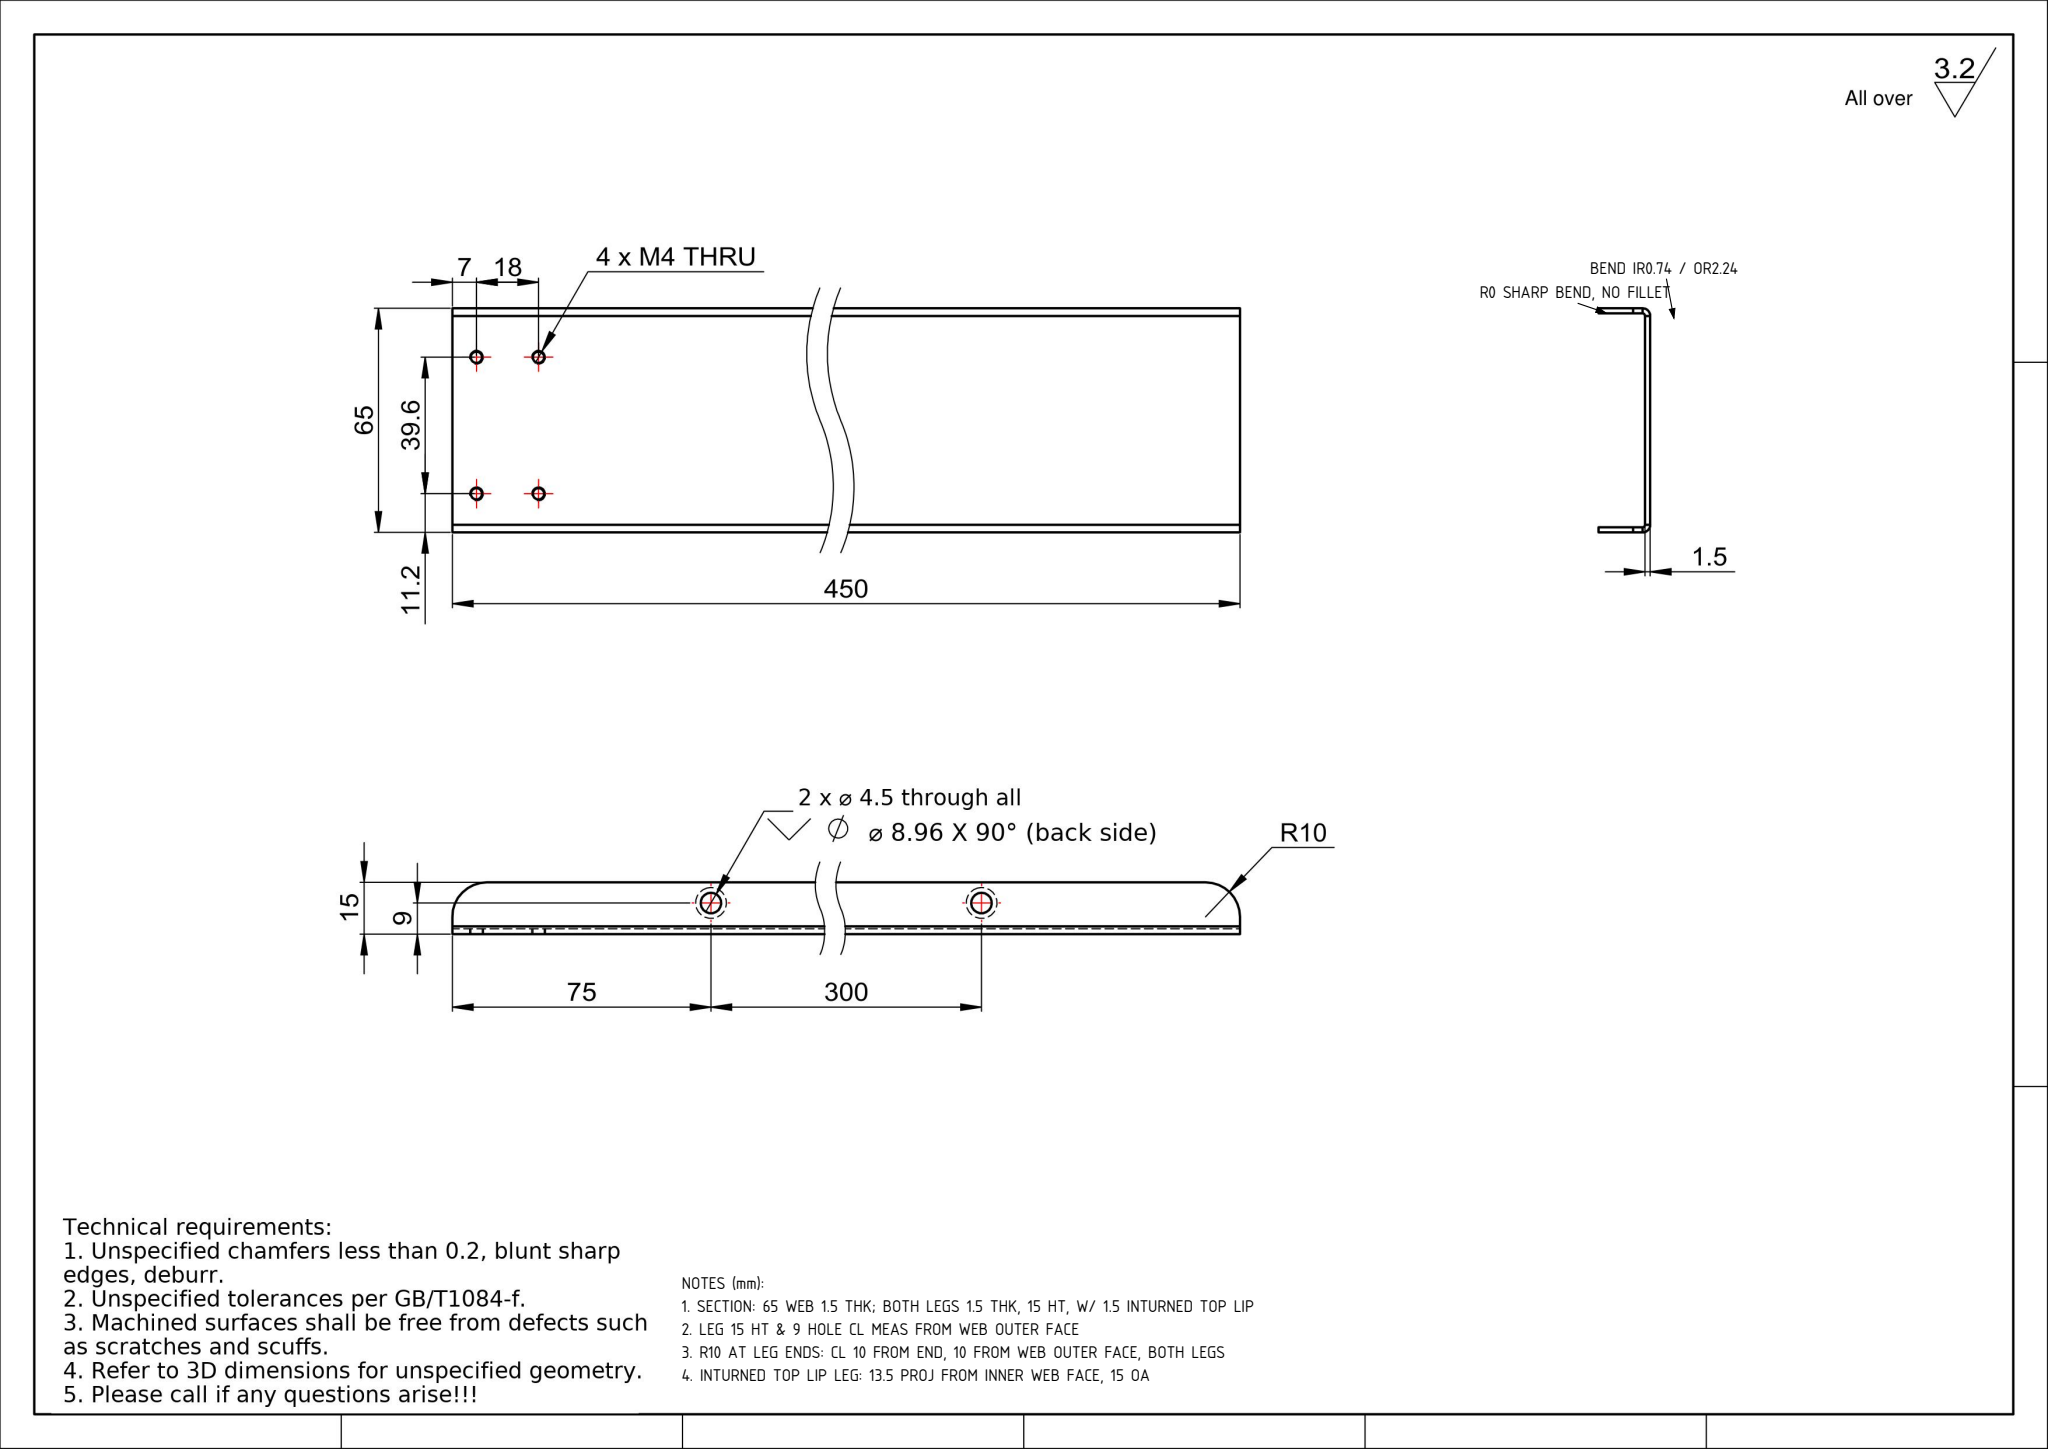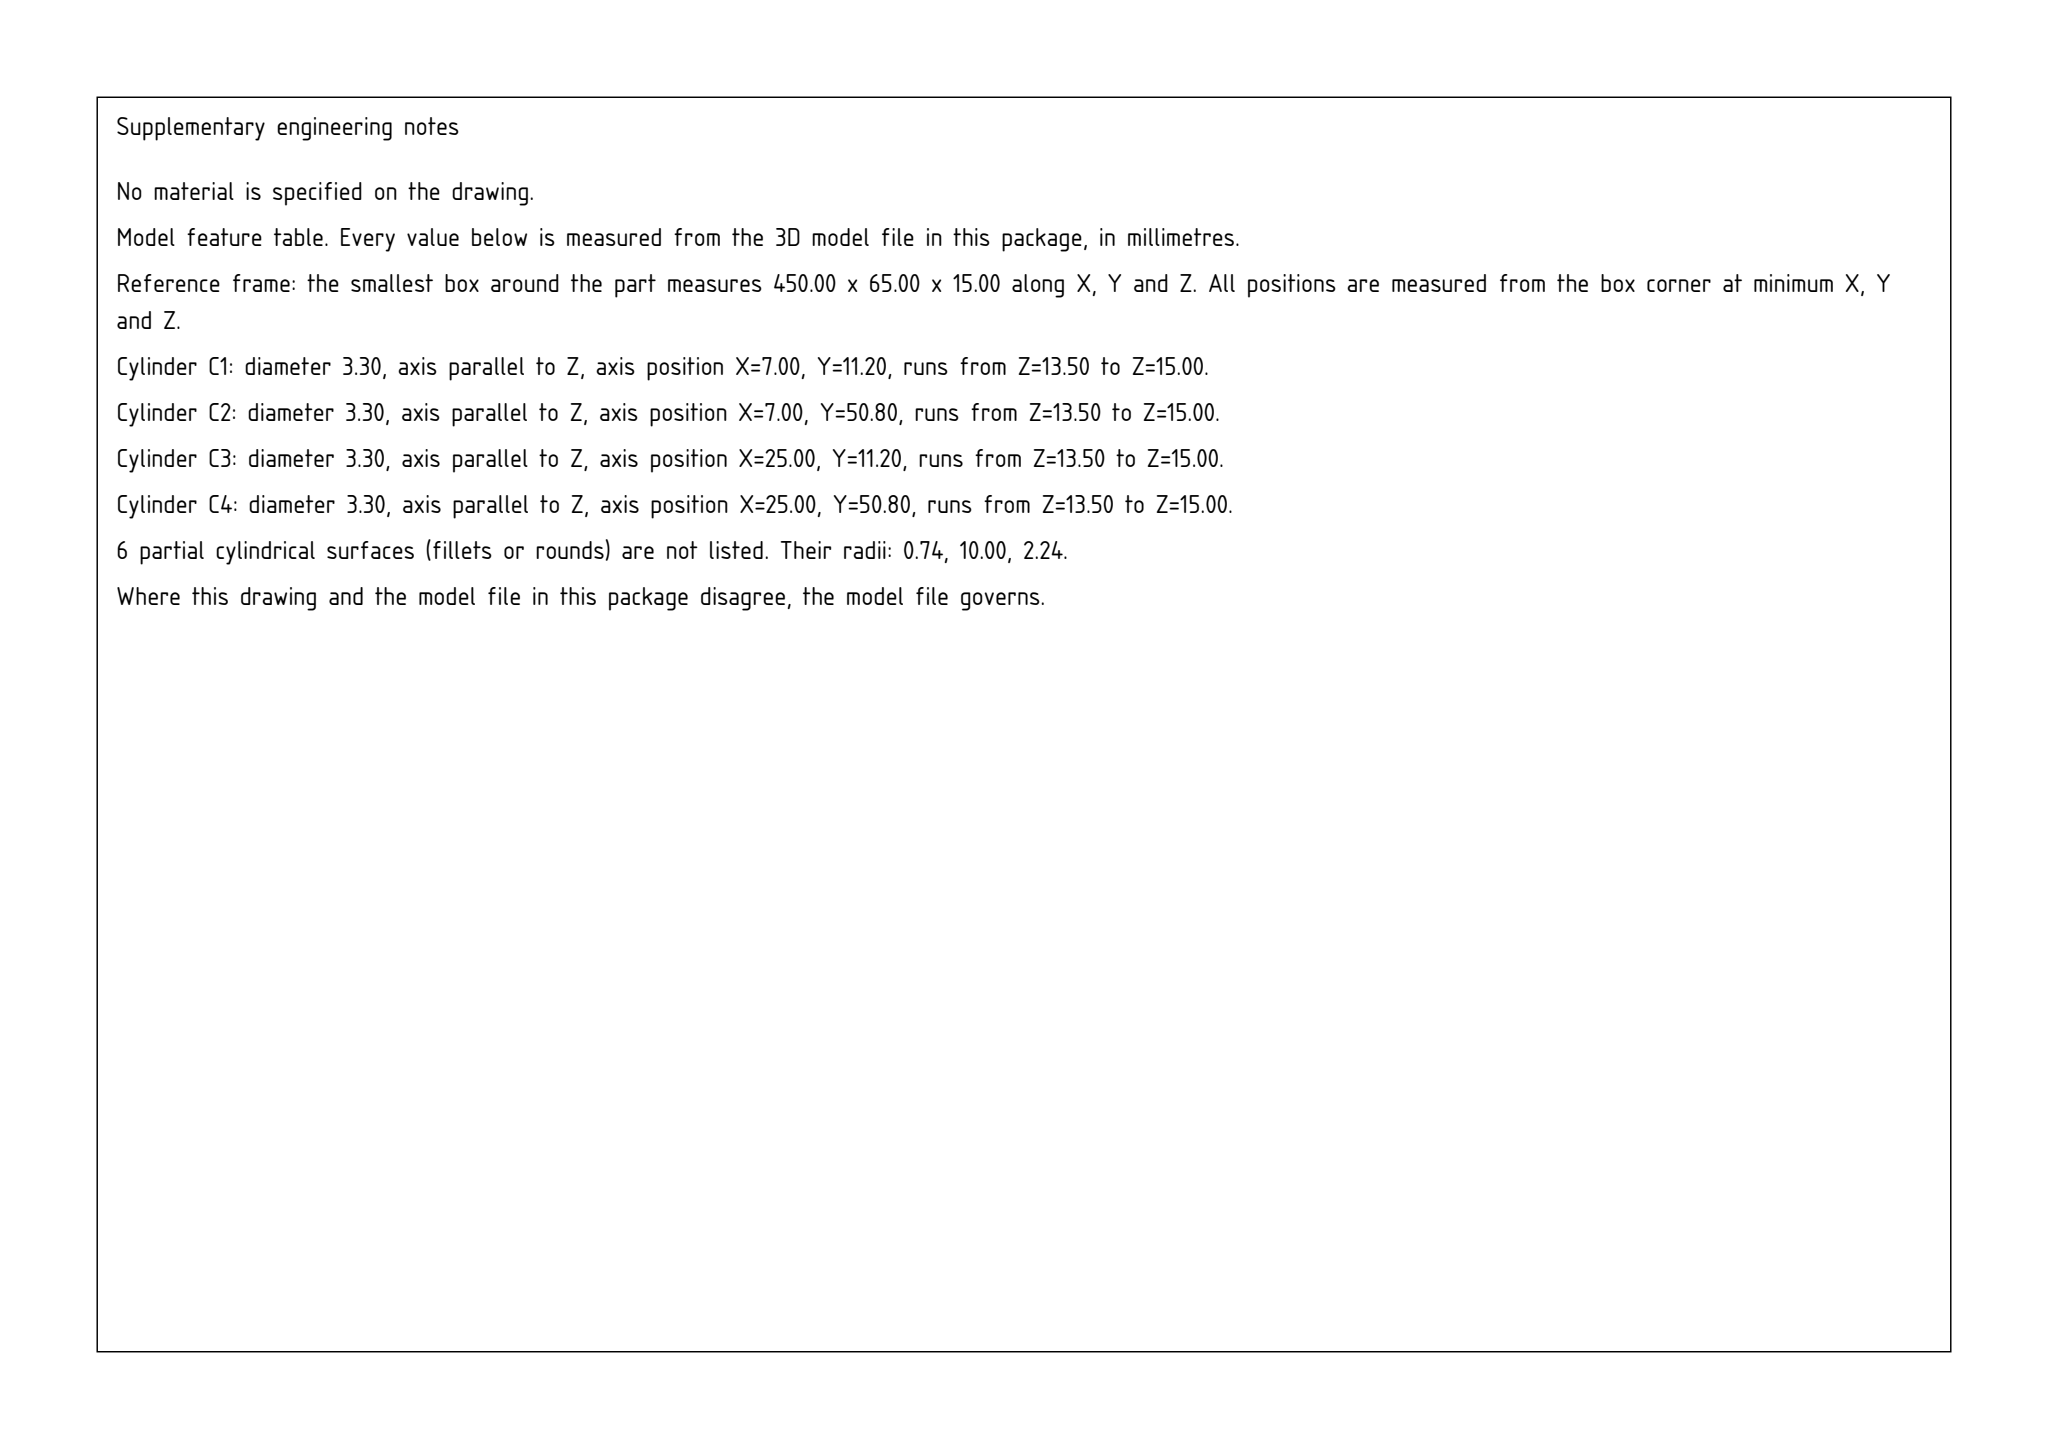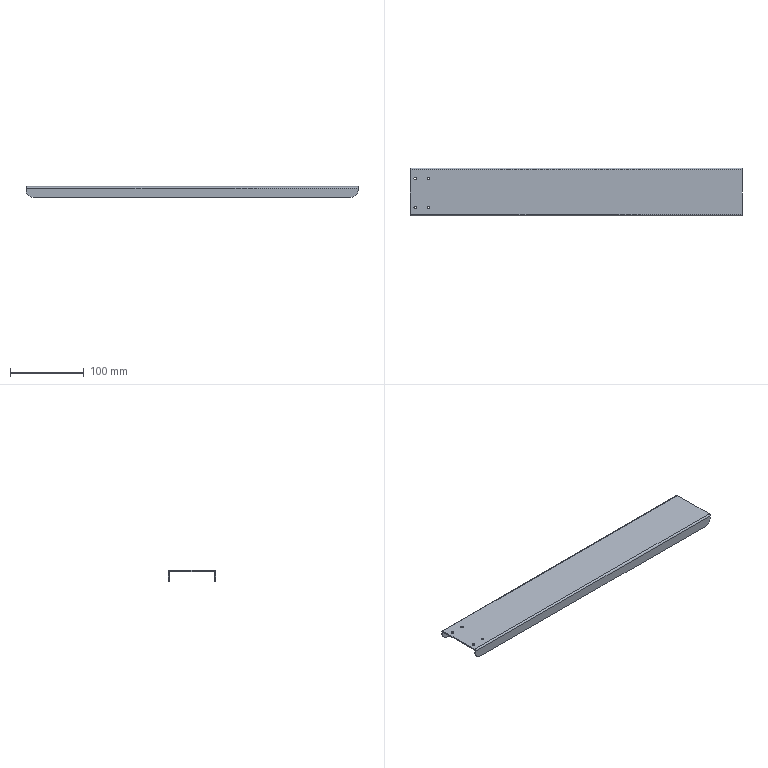Part | SolidWorks | mm | 1 solid | 38 faces | box 450 x 65 x 15 mm | volume 60926 mm3 | plane 18 | cylinder 16 | cone 4 | commonest cylinder face diameters 3.3 x8 20 x4 4.473 x2 1.473 x2
Drawing notes:
SECTION: 65 WEB 1.5 THK; BOTH LEGS 1.5 THK, 15 HT, W/ 1.5 INTURNED TOP LIP | from the solid: Y-planes 0/1.5 & 63.5/65 (1.5 thk legs); Z-planes 0, 13.5, 15; bbox 450x65x15
LEG 15 HT & 9 HOLE CL MEAS FROM WEB OUTER FACE | from the solid: Z-planes 0/15 give leg ht from web outer face at Z0; holes at z=9
LEG TO WEB BEND SHARP, R0 (NO FILLET) | from the solid: fillet_radii empty; y=0/1.5/63.5/65 meet z=0 planes, no cylinder at junction
LEG TO TOP LIP BEND IR0.74 / OR2.24, FULL 450 LG | from the solid: X-axis cyls Ø1.473 (R0.736) & Ø4.473 (R2.236) at y=2.24/62.76, z=12.76, len 450
R10 AT LEG ENDS: CL 10 FROM END, 10 FROM WEB OUTER FACE, BOTH LEGS | from the solid: cyl Ø20 axis Y at x=10 & 440, z=10, len 1.5 (both legs)
INTURNED TOP LIP LEG: 13.5 PROJ FROM INNER WEB FACE, 15 OA | from the solid: Lip walls y 0-1.5 & 63.5-65 run z 0 to web inner face z=13.5; bbox z=15 (web 1.5 thk, z 13.5-15)